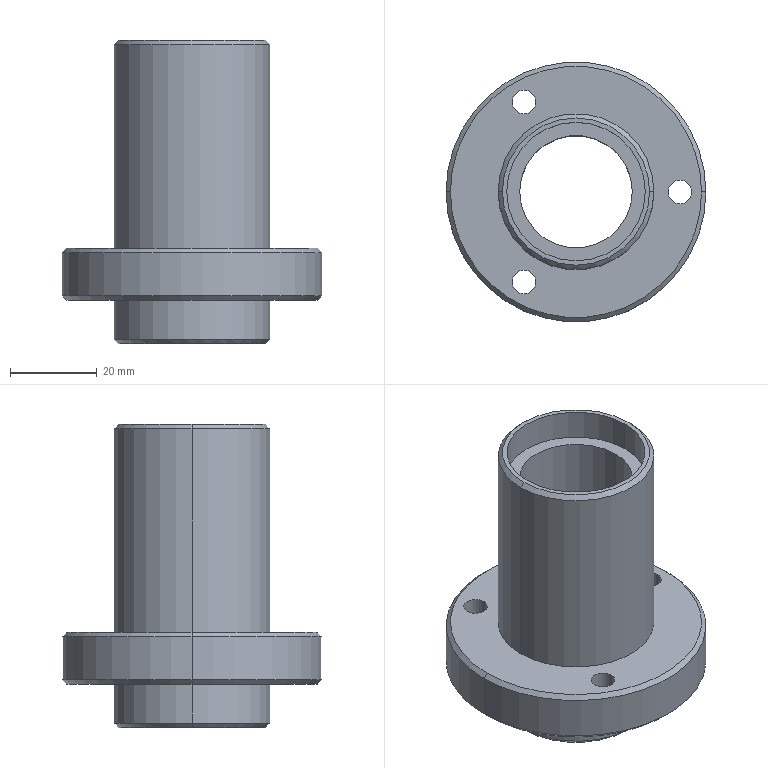Component | SolidWorks | JYTBJ-HeaderPlateFlangeSeatA-1 | 1 solid | 32 faces | box 60 x 60 x 70 mm | volume 50822 mm3 | cylinder 18 | cone 8 | plane 6 | commonest cylinder face diameters 5.5 x6 32 x4 36 x4 26 x2 60 x2
build123d program:
from build123d import *

# Parameters (mm, degrees)
F_5_5_5_5_DIAMETER_HOLE1_D = 5.5
CIRPATTERN1_COUNT          = 3
CHAMFER1_SIZE              = 1


with BuildPart() as part:
    # Sketch1 → Revolve1 (revolve)
    with BuildSketch(Plane.XY, mode=Mode.PRIVATE) as revolve1_sk:
        Polygon((16, 0), (18, 0), (18, 48), (30, 48), (30, 60), (18, 60), (18, 70), (16, 70), (16, 63), (13, 63), (13, 7), (16, 7), align=None)
    revolve(revolve1_sk.sketch.rotate(Axis((0, 0, 0), (0, 1, 0)), 90), axis=Axis((0, 0, 0), (0, 1, 0)))

    # 5.5 _5.5_ Diameter Hole1 (through all)
    with Locations(Plane.XZ.offset(-48)):
        with Locations((0, 24)):
            f_5_5_5_5_diameter_hole1 = Hole(F_5_5_5_5_DIAMETER_HOLE1_D / 2)

    # CirPattern1: 5.5 _5.5_ Diameter Hole1 ×3 about axis
    cirpattern1_axis = Axis((0, 0, 0), (0, 1, 0))
    for i in range(1, CIRPATTERN1_COUNT):
        add(f_5_5_5_5_diameter_hole1.rotate(cirpattern1_axis, i * 360 / CIRPATTERN1_COUNT), mode=Mode.SUBTRACT)

    # Chamfer1
    chamfer1_edges = [part.edges().sort_by_distance(p)[0] for p in [
        (0, 70, 18),
        (0, 60, 30),
        (0, 48, 30),
        (0, 0, 18),
    ]]
    chamfer(chamfer1_edges, length=CHAMFER1_SIZE)


solid = part.part

# Placed as in the assembly
solid = solid.moved(Location((3.373, 96.878, 42), (-90, 90, 0)))
STEP:
#1=COLOUR_RGB('',0.7922,0.8196,0.9333);
#2=FILL_AREA_STYLE_COLOUR('',#1);
#3=FILL_AREA_STYLE('',(#2));
#4=SURFACE_STYLE_FILL_AREA(#3);
#5=SURFACE_SIDE_STYLE('',(#4));
#6=SURFACE_STYLE_USAGE(.BOTH.,#5);
#7=PRESENTATION_STYLE_ASSIGNMENT((#6));
#8=CARTESIAN_POINT('',(-0.5365,3.814,1.654));
#9=VERTEX_POINT('',#8);
#10=CARTESIAN_POINT('',(0.8021,3.814,1.654));
#11=VERTEX_POINT('',#10);
#12=CARTESIAN_POINT('',(0.1328,3.814,1.654));
#13=DIRECTION('',(0.,0.,1.));
#14=DIRECTION('',(-1.,0.,0.));
#15=AXIS2_PLACEMENT_3D('',#12,#13,#14);
#16=CIRCLE('',#15,0.6693);
#17=EDGE_CURVE('',#9,#11,#16,.T.);
#18=ORIENTED_EDGE('',*,*,#17,.F.);
#19=CARTESIAN_POINT('',(-0.5759,3.814,1.614));
#20=VERTEX_POINT('',#19);
#21=CARTESIAN_POINT('',(-0.5365,3.814,1.654));
#22=DIRECTION('',(-0.7071,-0.,-0.7071));
#23=VECTOR('',#22,39.37);
#24=LINE('',#21,#23);
#25=EDGE_CURVE('',#9,#20,#24,.T.);
#26=ORIENTED_EDGE('',*,*,#25,.T.);
#27=CARTESIAN_POINT('',(0.8415,3.814,1.614));
#28=VERTEX_POINT('',#27);
#29=CARTESIAN_POINT('',(0.1328,3.814,1.614));
#30=DIRECTION('',(0.,0.,-1.));
#31=DIRECTION('',(-1.,0.,0.));
#32=AXIS2_PLACEMENT_3D('',#29,#30,#31);
#33=CIRCLE('',#32,0.7087);
#34=EDGE_CURVE('',#28,#20,#33,.T.);
#35=ORIENTED_EDGE('',*,*,#34,.F.);
#36=CARTESIAN_POINT('',(0.8021,3.814,1.654));
#37=DIRECTION('',(0.7071,-0.,-0.7071));
#38=VECTOR('',#37,39.37);
#39=LINE('',#36,#38);
#40=EDGE_CURVE('',#11,#28,#39,.T.);
#41=ORIENTED_EDGE('',*,*,#40,.F.);
#42=EDGE_LOOP('',(#18,#26,#35,#41));
#43=FACE_OUTER_BOUND('',#42,.T.);
#44=CARTESIAN_POINT('',(0.1328,3.814,1.654));
#45=DIRECTION('',(0.,0.,-1.));
#46=DIRECTION('',(1.,0.,0.));
#47=AXIS2_PLACEMENT_3D('',#44,#45,#46);
#48=CONICAL_SURFACE('',#47,0.6693,0.7854);
#49=ADVANCED_FACE('',(#43),#48,.T.);
#50=CARTESIAN_POINT('',(-1.009,3.814,-0.2362));
#51=VERTEX_POINT('',#50);
#52=CARTESIAN_POINT('',(1.275,3.814,-0.2362));
#53=VERTEX_POINT('',#52);
#54=CARTESIAN_POINT('',(0.1328,3.814,-0.2362));
#55=DIRECTION('',(0.,0.,1.));
#56=DIRECTION('',(-1.,0.,0.));
#57=AXIS2_PLACEMENT_3D('',#54,#55,#56);
#58=CIRCLE('',#57,1.142);
#59=EDGE_CURVE('',#51,#53,#58,.T.);
#60=ORIENTED_EDGE('',*,*,#59,.F.);
#61=CARTESIAN_POINT('',(-1.048,3.814,-0.2756));
#62=VERTEX_POINT('',#61);
#63=CARTESIAN_POINT('',(-1.009,3.814,-0.2362));
#64=DIRECTION('',(-0.7071,-0.,-0.7071));
#65=VECTOR('',#64,39.37);
#66=LINE('',#63,#65);
#67=EDGE_CURVE('',#51,#62,#66,.T.);
#68=ORIENTED_EDGE('',*,*,#67,.T.);
#69=CARTESIAN_POINT('',(1.314,3.814,-0.2756));
#70=VERTEX_POINT('',#69);
#71=CARTESIAN_POINT('',(0.1328,3.814,-0.2756));
#72=DIRECTION('',(0.,0.,-1.));
#73=DIRECTION('',(-1.,0.,0.));
#74=AXIS2_PLACEMENT_3D('',#71,#72,#73);
#75=CIRCLE('',#74,1.181);
#76=EDGE_CURVE('',#70,#62,#75,.T.);
#77=ORIENTED_EDGE('',*,*,#76,.F.);
#78=CARTESIAN_POINT('',(1.275,3.814,-0.2362));
#79=DIRECTION('',(0.7071,-0.,-0.7071));
#80=VECTOR('',#79,39.37);
#81=LINE('',#78,#80);
#82=EDGE_CURVE('',#53,#70,#81,.T.);
#83=ORIENTED_EDGE('',*,*,#82,.F.);
#84=EDGE_LOOP('',(#60,#68,#77,#83));
#85=FACE_OUTER_BOUND('',#84,.T.);
#86=CARTESIAN_POINT('',(0.1328,3.814,-0.2362));
#87=DIRECTION('',(0.,0.,-1.));
#88=DIRECTION('',(1.,0.,0.));
#89=AXIS2_PLACEMENT_3D('',#86,#87,#88);
#90=CONICAL_SURFACE('',#89,1.142,0.7854);
#91=ADVANCED_FACE('',(#85),#90,.T.);
#92=CARTESIAN_POINT('',(1.275,3.814,-0.7087));
#93=VERTEX_POINT('',#92);
#94=CARTESIAN_POINT('',(-1.009,3.814,-0.7087));
#95=VERTEX_POINT('',#94);
#96=CARTESIAN_POINT('',(0.1328,3.814,-0.7087));
#97=DIRECTION('',(0.,0.,-1.));
#98=DIRECTION('',(1.,0.,0.));
#99=AXIS2_PLACEMENT_3D('',#96,#97,#98);
#100=CIRCLE('',#99,1.142);
#101=EDGE_CURVE('',#93,#95,#100,.T.);
#102=ORIENTED_EDGE('',*,*,#101,.F.);
#103=CARTESIAN_POINT('',(1.314,3.814,-0.6693));
#104=VERTEX_POINT('',#103);
#105=CARTESIAN_POINT('',(1.314,3.814,-0.6693));
#106=DIRECTION('',(0.7071,-0.,0.7071));
#107=VECTOR('',#106,39.37);
#108=LINE('',#105,#107);
#109=EDGE_CURVE('',#93,#104,#108,.T.);
#110=ORIENTED_EDGE('',*,*,#109,.T.);
#111=CARTESIAN_POINT('',(-1.048,3.814,-0.6693));
#112=VERTEX_POINT('',#111);
#113=CARTESIAN_POINT('',(0.1328,3.814,-0.6693));
#114=DIRECTION('',(0.,0.,1.));
#115=DIRECTION('',(1.,0.,0.));
#116=AXIS2_PLACEMENT_3D('',#113,#114,#115);
#117=CIRCLE('',#116,1.181);
#118=EDGE_CURVE('',#112,#104,#117,.T.);
#119=ORIENTED_EDGE('',*,*,#118,.F.);
#120=CARTESIAN_POINT('',(-1.048,3.814,-0.6693));
#121=DIRECTION('',(-0.7071,0.,0.7071));
#122=VECTOR('',#121,39.37);
#123=LINE('',#120,#122);
#124=EDGE_CURVE('',#95,#112,#123,.T.);
#125=ORIENTED_EDGE('',*,*,#124,.F.);
#126=EDGE_LOOP('',(#102,#110,#119,#125));
#127=FACE_OUTER_BOUND('',#126,.T.);
#128=CARTESIAN_POINT('',(0.1328,3.814,-0.6693));
#129=DIRECTION('',(0.,0.,1.));
#130=DIRECTION('',(-1.,0.,0.));
#131=AXIS2_PLACEMENT_3D('',#128,#129,#130);
#132=CONICAL_SURFACE('',#131,1.181,0.7854);
#133=ADVANCED_FACE('',(#127),#132,.T.);
#134=CARTESIAN_POINT('',(0.8021,3.814,-1.102));
#135=VERTEX_POINT('',#134);
#136=CARTESIAN_POINT('',(-0.5365,3.814,-1.102));
#137=VERTEX_POINT('',#136);
#138=CARTESIAN_POINT('',(0.1328,3.814,-1.102));
#139=DIRECTION('',(0.,0.,-1.));
#140=DIRECTION('',(1.,0.,0.));
#141=AXIS2_PLACEMENT_3D('',#138,#139,#140);
#142=CIRCLE('',#141,0.6693);
#143=EDGE_CURVE('',#135,#137,#142,.T.);
#144=ORIENTED_EDGE('',*,*,#143,.F.);
#145=CARTESIAN_POINT('',(0.8415,3.814,-1.063));
#146=VERTEX_POINT('',#145);
#147=CARTESIAN_POINT('',(0.8415,3.814,-1.063));
#148=DIRECTION('',(0.7071,-0.,0.7071));
#149=VECTOR('',#148,39.37);
#150=LINE('',#147,#149);
#151=EDGE_CURVE('',#135,#146,#150,.T.);
#152=ORIENTED_EDGE('',*,*,#151,.T.);
#153=CARTESIAN_POINT('',(-0.5759,3.814,-1.063));
#154=VERTEX_POINT('',#153);
#155=CARTESIAN_POINT('',(0.1328,3.814,-1.063));
#156=DIRECTION('',(0.,0.,1.));
#157=DIRECTION('',(1.,0.,0.));
#158=AXIS2_PLACEMENT_3D('',#155,#156,#157);
#159=CIRCLE('',#158,0.7087);
#160=EDGE_CURVE('',#154,#146,#159,.T.);
#161=ORIENTED_EDGE('',*,*,#160,.F.);
#162=CARTESIAN_POINT('',(-0.5759,3.814,-1.063));
#163=DIRECTION('',(-0.7071,0.,0.7071));
#164=VECTOR('',#163,39.37);
#165=LINE('',#162,#164);
#166=EDGE_CURVE('',#137,#154,#165,.T.);
#167=ORIENTED_EDGE('',*,*,#166,.F.);
#168=EDGE_LOOP('',(#144,#152,#161,#167));
#169=FACE_OUTER_BOUND('',#168,.T.);
#170=CARTESIAN_POINT('',(0.1328,3.814,-1.063));
#171=DIRECTION('',(0.,0.,1.));
#172=DIRECTION('',(-1.,0.,0.));
#173=AXIS2_PLACEMENT_3D('',#170,#171,#172);
#174=CONICAL_SURFACE('',#173,0.7087,0.7854);
#175=ADVANCED_FACE('',(#169),#174,.T.);
#176=CARTESIAN_POINT('',(-0.4479,2.996,-0.7087));
#177=VERTEX_POINT('',#176);
#178=CARTESIAN_POINT('',(-0.2314,2.996,-0.7087));
#179=VERTEX_POINT('',#178);
#180=CARTESIAN_POINT('',(-0.3396,2.996,-0.7087));
#181=DIRECTION('',(0.,0.,-1.));
#182=DIRECTION('',(1.,0.,0.));
#183=AXIS2_PLACEMENT_3D('',#180,#181,#182);
#184=CIRCLE('',#183,0.1083);
#185=EDGE_CURVE('',#177,#179,#184,.T.);
#186=ORIENTED_EDGE('',*,*,#185,.T.);
#187=CARTESIAN_POINT('',(-0.2314,2.996,-0.2362));
#188=VERTEX_POINT('',#187);
#189=CARTESIAN_POINT('',(-0.2314,2.996,-0.2362));
#190=DIRECTION('',(0.,0.,1.));
#191=VECTOR('',#190,39.37);
#192=LINE('',#189,#191);
#193=EDGE_CURVE('',#179,#188,#192,.T.);
#194=ORIENTED_EDGE('',*,*,#193,.T.);
#195=CARTESIAN_POINT('',(-0.4479,2.996,-0.2362));
#196=VERTEX_POINT('',#195);
#197=CARTESIAN_POINT('',(-0.3396,2.996,-0.2362));
#198=DIRECTION('',(0.,0.,1.));
#199=DIRECTION('',(-1.,0.,0.));
#200=AXIS2_PLACEMENT_3D('',#197,#198,#199);
#201=CIRCLE('',#200,0.1083);
#202=EDGE_CURVE('',#188,#196,#201,.T.);
#203=ORIENTED_EDGE('',*,*,#202,.T.);
#204=CARTESIAN_POINT('',(-0.4479,2.996,-0.2362));
#205=DIRECTION('',(0.,0.,1.));
#206=VECTOR('',#205,39.37);
#207=LINE('',#204,#206);
#208=EDGE_CURVE('',#177,#196,#207,.T.);
#209=ORIENTED_EDGE('',*,*,#208,.F.);
#210=EDGE_LOOP('',(#186,#194,#203,#209));
#211=FACE_OUTER_BOUND('',#210,.T.);
#212=CARTESIAN_POINT('',(-0.3396,2.996,-0.2362));
#213=DIRECTION('',(0.,0.,1.));
#214=DIRECTION('',(-1.,0.,0.));
#215=AXIS2_PLACEMENT_3D('',#212,#213,#214);
#216=CYLINDRICAL_SURFACE('',#215,0.1083);
#217=ADVANCED_FACE('',(#211),#216,.F.);
#218=CARTESIAN_POINT('',(-0.4479,4.632,-0.7087));
#219=VERTEX_POINT('',#218);
#220=CARTESIAN_POINT('',(-0.2314,4.632,-0.7087));
#221=VERTEX_POINT('',#220);
#222=CARTESIAN_POINT('',(-0.3396,4.632,-0.7087));
#223=DIRECTION('',(0.,0.,-1.));
#224=DIRECTION('',(1.,0.,0.));
#225=AXIS2_PLACEMENT_3D('',#222,#223,#224);
#226=CIRCLE('',#225,0.1083);
#227=EDGE_CURVE('',#219,#221,#226,.T.);
#228=ORIENTED_EDGE('',*,*,#227,.T.);
#229=CARTESIAN_POINT('',(-0.2314,4.632,-0.2362));
#230=VERTEX_POINT('',#229);
#231=CARTESIAN_POINT('',(-0.2314,4.632,-0.2362));
#232=DIRECTION('',(0.,0.,1.));
#233=VECTOR('',#232,39.37);
#234=LINE('',#231,#233);
#235=EDGE_CURVE('',#221,#230,#234,.T.);
#236=ORIENTED_EDGE('',*,*,#235,.T.);
#237=CARTESIAN_POINT('',(-0.4479,4.632,-0.2362));
#238=VERTEX_POINT('',#237);
#239=CARTESIAN_POINT('',(-0.3396,4.632,-0.2362));
#240=DIRECTION('',(0.,0.,1.));
#241=DIRECTION('',(-1.,0.,0.));
#242=AXIS2_PLACEMENT_3D('',#239,#240,#241);
#243=CIRCLE('',#242,0.1083);
#244=EDGE_CURVE('',#230,#238,#243,.T.);
#245=ORIENTED_EDGE('',*,*,#244,.T.);
#246=CARTESIAN_POINT('',(-0.4479,4.632,-0.2362));
#247=DIRECTION('',(0.,0.,1.));
#248=VECTOR('',#247,39.37);
#249=LINE('',#246,#248);
#250=EDGE_CURVE('',#219,#238,#249,.T.);
#251=ORIENTED_EDGE('',*,*,#250,.F.);
#252=EDGE_LOOP('',(#228,#236,#245,#251));
#253=FACE_OUTER_BOUND('',#252,.T.);
#254=CARTESIAN_POINT('',(-0.3396,4.632,-0.2362));
#255=DIRECTION('',(0.,0.,1.));
#256=DIRECTION('',(-1.,0.,0.));
#257=AXIS2_PLACEMENT_3D('',#254,#255,#256);
#258=CYLINDRICAL_SURFACE('',#257,0.1083);
#259=ADVANCED_FACE('',(#253),#258,.F.);
#260=CARTESIAN_POINT('',(0.9694,3.814,-0.7087));
#261=VERTEX_POINT('',#260);
#262=CARTESIAN_POINT('',(1.186,3.814,-0.7087));
#263=VERTEX_POINT('',#262);
#264=CARTESIAN_POINT('',(1.078,3.814,-0.7087));
#265=DIRECTION('',(0.,0.,-1.));
#266=DIRECTION('',(1.,0.,0.));
#267=AXIS2_PLACEMENT_3D('',#264,#265,#266);
#268=CIRCLE('',#267,0.1083);
#269=EDGE_CURVE('',#261,#263,#268,.T.);
#270=ORIENTED_EDGE('',*,*,#269,.T.);
#271=CARTESIAN_POINT('',(1.186,3.814,-0.2362));
#272=VERTEX_POINT('',#271);
#273=CARTESIAN_POINT('',(1.186,3.814,-0.2362));
#274=DIRECTION('',(0.,0.,1.));
#275=VECTOR('',#274,39.37);
#276=LINE('',#273,#275);
#277=EDGE_CURVE('',#263,#272,#276,.T.);
#278=ORIENTED_EDGE('',*,*,#277,.T.);
#279=CARTESIAN_POINT('',(0.9694,3.814,-0.2362));
#280=VERTEX_POINT('',#279);
#281=CARTESIAN_POINT('',(1.078,3.814,-0.2362));
#282=DIRECTION('',(0.,0.,1.));
#283=DIRECTION('',(-1.,0.,0.));
#284=AXIS2_PLACEMENT_3D('',#281,#282,#283);
#285=CIRCLE('',#284,0.1083);
#286=EDGE_CURVE('',#272,#280,#285,.T.);
#287=ORIENTED_EDGE('',*,*,#286,.T.);
#288=CARTESIAN_POINT('',(0.9694,3.814,-0.2362));
#289=DIRECTION('',(0.,0.,1.));
#290=VECTOR('',#289,39.37);
#291=LINE('',#288,#290);
#292=EDGE_CURVE('',#261,#280,#291,.T.);
#293=ORIENTED_EDGE('',*,*,#292,.F.);
#294=EDGE_LOOP('',(#270,#278,#287,#293));
#295=FACE_OUTER_BOUND('',#294,.T.);
#296=CARTESIAN_POINT('',(1.078,3.814,-0.2362));
#297=DIRECTION('',(0.,0.,1.));
#298=DIRECTION('',(-1.,0.,0.));
#299=AXIS2_PLACEMENT_3D('',#296,#297,#298);
#300=CYLINDRICAL_SURFACE('',#299,0.1083);
#301=ADVANCED_FACE('',(#295),#300,.F.);
#302=CARTESIAN_POINT('',(0.6446,3.814,-0.8268));
#303=VERTEX_POINT('',#302);
#304=CARTESIAN_POINT('',(-0.379,3.814,-0.8268));
#305=VERTEX_POINT('',#304);
#306=CARTESIAN_POINT('',(0.1328,3.814,-0.8268));
#307=DIRECTION('',(0.,0.,1.));
#308=DIRECTION('',(-1.,0.,0.));
#309=AXIS2_PLACEMENT_3D('',#306,#307,#308);
#310=CIRCLE('',#309,0.5118);
#311=EDGE_CURVE('',#303,#305,#310,.T.);
#312=ORIENTED_EDGE('',*,*,#311,.F.);
#313=CARTESIAN_POINT('',(0.6446,3.814,1.378));
#314=VERTEX_POINT('',#313);
#315=CARTESIAN_POINT('',(0.6446,3.814,1.654));
#316=DIRECTION('',(0.,0.,1.));
#317=VECTOR('',#316,39.37);
#318=LINE('',#315,#317);
#319=EDGE_CURVE('',#303,#314,#318,.T.);
#320=ORIENTED_EDGE('',*,*,#319,.T.);
#321=CARTESIAN_POINT('',(-0.379,3.814,1.378));
#322=VERTEX_POINT('',#321);
#323=CARTESIAN_POINT('',(0.1328,3.814,1.378));
#324=DIRECTION('',(0.,0.,1.));
#325=DIRECTION('',(-1.,0.,0.));
#326=AXIS2_PLACEMENT_3D('',#323,#324,#325);
#327=CIRCLE('',#326,0.5118);
#328=EDGE_CURVE('',#314,#322,#327,.T.);
#329=ORIENTED_EDGE('',*,*,#328,.T.);
#330=CARTESIAN_POINT('',(-0.379,3.814,1.654));
#331=DIRECTION('',(0.,0.,1.));
#332=VECTOR('',#331,39.37);
#333=LINE('',#330,#332);
#334=EDGE_CURVE('',#305,#322,#333,.T.);
#335=ORIENTED_EDGE('',*,*,#334,.F.);
#336=EDGE_LOOP('',(#312,#320,#329,#335));
#337=FACE_OUTER_BOUND('',#336,.T.);
#338=CARTESIAN_POINT('',(0.1328,3.814,1.654));
#339=DIRECTION('',(0.,0.,1.));
#340=DIRECTION('',(-1.,0.,0.));
#341=AXIS2_PLACEMENT_3D('',#338,#339,#340);
#342=CYLINDRICAL_SURFACE('',#341,0.5118);
#343=ADVANCED_FACE('',(#337),#342,.F.);
#344=CARTESIAN_POINT('',(0.7627,3.814,-1.102));
#345=VERTEX_POINT('',#344);
#346=CARTESIAN_POINT('',(-0.4971,3.814,-1.102));
#347=VERTEX_POINT('',#346);
#348=CARTESIAN_POINT('',(0.1328,3.814,-1.102));
#349=DIRECTION('',(0.,0.,1.));
#350=DIRECTION('',(-1.,0.,0.));
#351=AXIS2_PLACEMENT_3D('',#348,#349,#350);
#352=CIRCLE('',#351,0.6299);
#353=EDGE_CURVE('',#345,#347,#352,.T.);
#354=ORIENTED_EDGE('',*,*,#353,.F.);
#355=CARTESIAN_POINT('',(0.7627,3.814,-0.8268));
#356=VERTEX_POINT('',#355);
#357=CARTESIAN_POINT('',(0.7627,3.814,1.654));
#358=DIRECTION('',(0.,0.,1.));
#359=VECTOR('',#358,39.37);
#360=LINE('',#357,#359);
#361=EDGE_CURVE('',#345,#356,#360,.T.);
#362=ORIENTED_EDGE('',*,*,#361,.T.);
#363=CARTESIAN_POINT('',(-0.4971,3.814,-0.8268));
#364=VERTEX_POINT('',#363);
#365=CARTESIAN_POINT('',(0.1328,3.814,-0.8268));
#366=DIRECTION('',(0.,0.,1.));
#367=DIRECTION('',(-1.,0.,0.));
#368=AXIS2_PLACEMENT_3D('',#365,#366,#367);
#369=CIRCLE('',#368,0.6299);
#370=EDGE_CURVE('',#356,#364,#369,.T.);
#371=ORIENTED_EDGE('',*,*,#370,.T.);
#372=CARTESIAN_POINT('',(-0.4971,3.814,1.654));
#373=DIRECTION('',(0.,0.,1.));
#374=VECTOR('',#373,39.37);
#375=LINE('',#372,#374);
#376=EDGE_CURVE('',#347,#364,#375,.T.);
#377=ORIENTED_EDGE('',*,*,#376,.F.);
#378=EDGE_LOOP('',(#354,#362,#371,#377));
#379=FACE_OUTER_BOUND('',#378,.T.);
#380=CARTESIAN_POINT('',(0.1328,3.814,1.654));
#381=DIRECTION('',(0.,0.,1.));
#382=DIRECTION('',(-1.,0.,0.));
#383=AXIS2_PLACEMENT_3D('',#380,#381,#382);
#384=CYLINDRICAL_SURFACE('',#383,0.6299);
#385=ADVANCED_FACE('',(#379),#384,.F.);
#386=ORIENTED_EDGE('',*,*,#160,.T.);
#387=CARTESIAN_POINT('',(0.8415,3.814,-0.7087));
#388=VERTEX_POINT('',#387);
#389=CARTESIAN_POINT('',(0.8415,3.814,1.654));
#390=DIRECTION('',(0.,0.,1.));
#391=VECTOR('',#390,39.37);
#392=LINE('',#389,#391);
#393=EDGE_CURVE('',#146,#388,#392,.T.);
#394=ORIENTED_EDGE('',*,*,#393,.T.);
#395=CARTESIAN_POINT('',(-0.5759,3.814,-0.7087));
#396=VERTEX_POINT('',#395);
#397=CARTESIAN_POINT('',(0.1328,3.814,-0.7087));
#398=DIRECTION('',(0.,0.,1.));
#399=DIRECTION('',(-1.,0.,0.));
#400=AXIS2_PLACEMENT_3D('',#397,#398,#399);
#401=CIRCLE('',#400,0.7087);
#402=EDGE_CURVE('',#396,#388,#401,.T.);
#403=ORIENTED_EDGE('',*,*,#402,.F.);
#404=CARTESIAN_POINT('',(-0.5759,3.814,1.654));
#405=DIRECTION('',(0.,0.,1.));
#406=VECTOR('',#405,39.37);
#407=LINE('',#404,#406);
#408=EDGE_CURVE('',#154,#396,#407,.T.);
#409=ORIENTED_EDGE('',*,*,#408,.F.);
#410=EDGE_LOOP('',(#386,#394,#403,#409));
#411=FACE_OUTER_BOUND('',#410,.T.);
#412=CARTESIAN_POINT('',(0.1328,3.814,1.654));
#413=DIRECTION('',(0.,0.,1.));
#414=DIRECTION('',(-1.,0.,0.));
#415=AXIS2_PLACEMENT_3D('',#412,#413,#414);
#416=CYLINDRICAL_SURFACE('',#415,0.7087);
#417=ADVANCED_FACE('',(#411),#416,.T.);
#418=ORIENTED_EDGE('',*,*,#118,.T.);
#419=CARTESIAN_POINT('',(1.314,3.814,1.654));
#420=DIRECTION('',(0.,0.,1.));
#421=VECTOR('',#420,39.37);
#422=LINE('',#419,#421);
#423=EDGE_CURVE('',#104,#70,#422,.T.);
#424=ORIENTED_EDGE('',*,*,#423,.T.);
#425=ORIENTED_EDGE('',*,*,#76,.T.);
#426=CARTESIAN_POINT('',(-1.048,3.814,1.654));
#427=DIRECTION('',(0.,0.,1.));
#428=VECTOR('',#427,39.37);
#429=LINE('',#426,#428);
#430=EDGE_CURVE('',#112,#62,#429,.T.);
#431=ORIENTED_EDGE('',*,*,#430,.F.);
#432=EDGE_LOOP('',(#418,#424,#425,#431));
#433=FACE_OUTER_BOUND('',#432,.T.);
#434=CARTESIAN_POINT('',(0.1328,3.814,1.654));
#435=DIRECTION('',(0.,0.,1.));
#436=DIRECTION('',(-1.,0.,0.));
#437=AXIS2_PLACEMENT_3D('',#434,#435,#436);
#438=CYLINDRICAL_SURFACE('',#437,1.181);
#439=ADVANCED_FACE('',(#433),#438,.T.);
#440=CARTESIAN_POINT('',(-0.5759,3.814,-0.2362));
#441=VERTEX_POINT('',#440);
#442=CARTESIAN_POINT('',(0.8415,3.814,-0.2362));
#443=VERTEX_POINT('',#442);
#444=CARTESIAN_POINT('',(0.1328,3.814,-0.2362));
#445=DIRECTION('',(0.,0.,1.));
#446=DIRECTION('',(-1.,0.,0.));
#447=AXIS2_PLACEMENT_3D('',#444,#445,#446);
#448=CIRCLE('',#447,0.7087);
#449=EDGE_CURVE('',#441,#443,#448,.T.);
#450=ORIENTED_EDGE('',*,*,#449,.T.);
#451=CARTESIAN_POINT('',(0.8415,3.814,1.654));
#452=DIRECTION('',(0.,0.,1.));
#453=VECTOR('',#452,39.37);
#454=LINE('',#451,#453);
#455=EDGE_CURVE('',#443,#28,#454,.T.);
#456=ORIENTED_EDGE('',*,*,#455,.T.);
#457=ORIENTED_EDGE('',*,*,#34,.T.);
#458=CARTESIAN_POINT('',(-0.5759,3.814,1.654));
#459=DIRECTION('',(0.,0.,1.));
#460=VECTOR('',#459,39.37);
#461=LINE('',#458,#460);
#462=EDGE_CURVE('',#441,#20,#461,.T.);
#463=ORIENTED_EDGE('',*,*,#462,.F.);
#464=EDGE_LOOP('',(#450,#456,#457,#463));
#465=FACE_OUTER_BOUND('',#464,.T.);
#466=CARTESIAN_POINT('',(0.1328,3.814,1.654));
#467=DIRECTION('',(0.,0.,1.));
#468=DIRECTION('',(-1.,0.,0.));
#469=AXIS2_PLACEMENT_3D('',#466,#467,#468);
#470=CYLINDRICAL_SURFACE('',#469,0.7087);
#471=ADVANCED_FACE('',(#465),#470,.T.);
#472=CARTESIAN_POINT('',(0.7627,3.814,1.378));
#473=VERTEX_POINT('',#472);
#474=CARTESIAN_POINT('',(-0.4971,3.814,1.378));
#475=VERTEX_POINT('',#474);
#476=CARTESIAN_POINT('',(0.1328,3.814,1.378));
#477=DIRECTION('',(0.,0.,1.));
#478=DIRECTION('',(-1.,0.,0.));
#479=AXIS2_PLACEMENT_3D('',#476,#477,#478);
#480=CIRCLE('',#479,0.6299);
#481=EDGE_CURVE('',#473,#475,#480,.T.);
#482=ORIENTED_EDGE('',*,*,#481,.F.);
#483=CARTESIAN_POINT('',(0.7627,3.814,1.654));
#484=VERTEX_POINT('',#483);
#485=CARTESIAN_POINT('',(0.7627,3.814,1.654));
#486=DIRECTION('',(0.,0.,1.));
#487=VECTOR('',#486,39.37);
#488=LINE('',#485,#487);
#489=EDGE_CURVE('',#473,#484,#488,.T.);
#490=ORIENTED_EDGE('',*,*,#489,.T.);
#491=CARTESIAN_POINT('',(-0.4971,3.814,1.654));
#492=VERTEX_POINT('',#491);
#493=CARTESIAN_POINT('',(0.1328,3.814,1.654));
#494=DIRECTION('',(0.,0.,1.));
#495=DIRECTION('',(-1.,0.,0.));
#496=AXIS2_PLACEMENT_3D('',#493,#494,#495);
#497=CIRCLE('',#496,0.6299);
#498=EDGE_CURVE('',#484,#492,#497,.T.);
#499=ORIENTED_EDGE('',*,*,#498,.T.);
#500=CARTESIAN_POINT('',(-0.4971,3.814,1.654));
#501=DIRECTION('',(0.,0.,1.));
#502=VECTOR('',#501,39.37);
#503=LINE('',#500,#502);
#504=EDGE_CURVE('',#475,#492,#503,.T.);
#505=ORIENTED_EDGE('',*,*,#504,.F.);
#506=EDGE_LOOP('',(#482,#490,#499,#505));
#507=FACE_OUTER_BOUND('',#506,.T.);
#508=CARTESIAN_POINT('',(0.1328,3.814,1.654));
#509=DIRECTION('',(0.,0.,1.));
#510=DIRECTION('',(-1.,0.,0.));
#511=AXIS2_PLACEMENT_3D('',#508,#509,#510);
#512=CYLINDRICAL_SURFACE('',#511,0.6299);
#513=ADVANCED_FACE('',(#507),#512,.F.);
#514=ORIENTED_EDGE('',*,*,#489,.F.);
#515=CARTESIAN_POINT('',(0.1328,3.814,1.378));
#516=DIRECTION('',(0.,0.,1.));
#517=DIRECTION('',(-1.,0.,0.));
#518=AXIS2_PLACEMENT_3D('',#515,#516,#517);
#519=CIRCLE('',#518,0.6299);
#520=EDGE_CURVE('',#475,#473,#519,.T.);
#521=ORIENTED_EDGE('',*,*,#520,.F.);
#522=ORIENTED_EDGE('',*,*,#504,.T.);
#523=CARTESIAN_POINT('',(0.1328,3.814,1.654));
#524=DIRECTION('',(0.,0.,1.));
#525=DIRECTION('',(-1.,0.,0.));
#526=AXIS2_PLACEMENT_3D('',#523,#524,#525);
#527=CIRCLE('',#526,0.6299);
#528=EDGE_CURVE('',#492,#484,#527,.T.);
#529=ORIENTED_EDGE('',*,*,#528,.T.);
#530=EDGE_LOOP('',(#514,#521,#522,#529));
#531=FACE_OUTER_BOUND('',#530,.T.);
#532=CARTESIAN_POINT('',(0.1328,3.814,1.654));
#533=DIRECTION('',(0.,0.,1.));
#534=DIRECTION('',(-1.,0.,0.));
#535=AXIS2_PLACEMENT_3D('',#532,#533,#534);
#536=CYLINDRICAL_SURFACE('',#535,0.6299);
#537=ADVANCED_FACE('',(#531),#536,.F.);
#538=CARTESIAN_POINT('',(0.1328,3.814,1.654));
#539=DIRECTION('',(0.,0.,1.));
#540=DIRECTION('',(-1.,0.,0.));
#541=AXIS2_PLACEMENT_3D('',#538,#539,#540);
#542=CIRCLE('',#541,0.6693);
#543=EDGE_CURVE('',#11,#9,#542,.T.);
#544=ORIENTED_EDGE('',*,*,#543,.T.);
#545=ORIENTED_EDGE('',*,*,#17,.T.);
#546=EDGE_LOOP('',(#544,#545));
#547=FACE_OUTER_BOUND('',#546,.T.);
#548=ORIENTED_EDGE('',*,*,#528,.F.);
#549=ORIENTED_EDGE('',*,*,#498,.F.);
#550=EDGE_LOOP('',(#548,#549));
#551=FACE_BOUND('',#550,.T.);
#552=CARTESIAN_POINT('',(0.1328,3.184,1.654));
#553=DIRECTION('',(0.,0.,1.));
#554=DIRECTION('',(-1.,0.,0.));
#555=AXIS2_PLACEMENT_3D('',#552,#553,#554);
#556=PLANE('',#555);
#557=ADVANCED_FACE('',(#547,#551),#556,.T.);
#558=ORIENTED_EDGE('',*,*,#455,.F.);
#559=CARTESIAN_POINT('',(0.1328,3.814,-0.2362));
#560=DIRECTION('',(0.,0.,1.));
#561=DIRECTION('',(-1.,0.,0.));
#562=AXIS2_PLACEMENT_3D('',#559,#560,#561);
#563=CIRCLE('',#562,0.7087);
#564=EDGE_CURVE('',#443,#441,#563,.T.);
#565=ORIENTED_EDGE('',*,*,#564,.T.);
#566=ORIENTED_EDGE('',*,*,#462,.T.);
#567=CARTESIAN_POINT('',(0.1328,3.814,1.614));
#568=DIRECTION('',(0.,0.,-1.));
#569=DIRECTION('',(-1.,0.,0.));
#570=AXIS2_PLACEMENT_3D('',#567,#568,#569);
#571=CIRCLE('',#570,0.7087);
#572=EDGE_CURVE('',#20,#28,#571,.T.);
#573=ORIENTED_EDGE('',*,*,#572,.T.);
#574=EDGE_LOOP('',(#558,#565,#566,#573));
#575=FACE_OUTER_BOUND('',#574,.T.);
#576=CARTESIAN_POINT('',(0.1328,3.814,1.654));
#577=DIRECTION('',(0.,0.,1.));
#578=DIRECTION('',(-1.,0.,0.));
#579=AXIS2_PLACEMENT_3D('',#576,#577,#578);
#580=CYLINDRICAL_SURFACE('',#579,0.7087);
#581=ADVANCED_FACE('',(#575),#580,.T.);
#582=CARTESIAN_POINT('',(0.1328,3.814,-0.2362));
#583=DIRECTION('',(0.,0.,1.));
#584=DIRECTION('',(-1.,0.,0.));
#585=AXIS2_PLACEMENT_3D('',#582,#583,#584);
#586=CIRCLE('',#585,1.142);
#587=EDGE_CURVE('',#53,#51,#586,.T.);
#588=ORIENTED_EDGE('',*,*,#587,.T.);
#589=ORIENTED_EDGE('',*,*,#59,.T.);
#590=EDGE_LOOP('',(#588,#589));
#591=FACE_OUTER_BOUND('',#590,.T.);
#592=CARTESIAN_POINT('',(-0.3396,2.996,-0.2362));
#593=DIRECTION('',(0.,0.,1.));
#594=DIRECTION('',(-1.,0.,0.));
#595=AXIS2_PLACEMENT_3D('',#592,#593,#594);
#596=CIRCLE('',#595,0.1083);
#597=EDGE_CURVE('',#196,#188,#596,.T.);
#598=ORIENTED_EDGE('',*,*,#597,.F.);
#599=ORIENTED_EDGE('',*,*,#202,.F.);
#600=EDGE_LOOP('',(#598,#599));
#601=FACE_BOUND('',#600,.T.);
#602=CARTESIAN_POINT('',(-0.3396,4.632,-0.2362));
#603=DIRECTION('',(0.,0.,1.));
#604=DIRECTION('',(-1.,0.,0.));
#605=AXIS2_PLACEMENT_3D('',#602,#603,#604);
#606=CIRCLE('',#605,0.1083);
#607=EDGE_CURVE('',#238,#230,#606,.T.);
#608=ORIENTED_EDGE('',*,*,#607,.F.);
#609=ORIENTED_EDGE('',*,*,#244,.F.);
#610=EDGE_LOOP('',(#608,#609));
#611=FACE_BOUND('',#610,.T.);
#612=CARTESIAN_POINT('',(1.078,3.814,-0.2362));
#613=DIRECTION('',(0.,0.,1.));
#614=DIRECTION('',(-1.,0.,0.));
#615=AXIS2_PLACEMENT_3D('',#612,#613,#614);
#616=CIRCLE('',#615,0.1083);
#617=EDGE_CURVE('',#280,#272,#616,.T.);
#618=ORIENTED_EDGE('',*,*,#617,.F.);
#619=ORIENTED_EDGE('',*,*,#286,.F.);
#620=EDGE_LOOP('',(#618,#619));
#621=FACE_BOUND('',#620,.T.);
#622=ORIENTED_EDGE('',*,*,#449,.F.);
#623=ORIENTED_EDGE('',*,*,#564,.F.);
#624=EDGE_LOOP('',(#622,#623));
#625=FACE_BOUND('',#624,.T.);
#626=CARTESIAN_POINT('',(0.1328,3.105,-0.2362));
#627=DIRECTION('',(0.,0.,1.));
#628=DIRECTION('',(-1.,0.,0.));
#629=AXIS2_PLACEMENT_3D('',#626,#627,#628);
#630=PLANE('',#629);
#631=ADVANCED_FACE('',(#591,#601,#611,#621,#625),#630,.T.);
#632=ORIENTED_EDGE('',*,*,#423,.F.);
#633=CARTESIAN_POINT('',(0.1328,3.814,-0.6693));
#634=DIRECTION('',(0.,0.,1.));
#635=DIRECTION('',(1.,0.,0.));
#636=AXIS2_PLACEMENT_3D('',#633,#634,#635);
#637=CIRCLE('',#636,1.181);
#638=EDGE_CURVE('',#104,#112,#637,.T.);
#639=ORIENTED_EDGE('',*,*,#638,.T.);
#640=ORIENTED_EDGE('',*,*,#430,.T.);
#641=CARTESIAN_POINT('',(0.1328,3.814,-0.2756));
#642=DIRECTION('',(0.,0.,-1.));
#643=DIRECTION('',(-1.,0.,0.));
#644=AXIS2_PLACEMENT_3D('',#641,#642,#643);
#645=CIRCLE('',#644,1.181);
#646=EDGE_CURVE('',#62,#70,#645,.T.);
#647=ORIENTED_EDGE('',*,*,#646,.T.);
#648=EDGE_LOOP('',(#632,#639,#640,#647));
#649=FACE_OUTER_BOUND('',#648,.T.);
#650=CARTESIAN_POINT('',(0.1328,3.814,1.654));
#651=DIRECTION('',(0.,0.,1.));
#652=DIRECTION('',(-1.,0.,0.));
#653=AXIS2_PLACEMENT_3D('',#650,#651,#652);
#654=CYLINDRICAL_SURFACE('',#653,1.181);
#655=ADVANCED_FACE('',(#649),#654,.T.);
#656=CARTESIAN_POINT('',(0.1328,3.814,-0.7087));
#657=DIRECTION('',(0.,0.,-1.));
#658=DIRECTION('',(1.,0.,0.));
#659=AXIS2_PLACEMENT_3D('',#656,#657,#658);
#660=CIRCLE('',#659,1.142);
#661=EDGE_CURVE('',#95,#93,#660,.T.);
#662=ORIENTED_EDGE('',*,*,#661,.T.);
#663=ORIENTED_EDGE('',*,*,#101,.T.);
#664=EDGE_LOOP('',(#662,#663));
#665=FACE_OUTER_BOUND('',#664,.T.);
#666=ORIENTED_EDGE('',*,*,#185,.F.);
#667=CARTESIAN_POINT('',(-0.3396,2.996,-0.7087));
#668=DIRECTION('',(0.,0.,-1.));
#669=DIRECTION('',(1.,0.,0.));
#670=AXIS2_PLACEMENT_3D('',#667,#668,#669);
#671=CIRCLE('',#670,0.1083);
#672=EDGE_CURVE('',#179,#177,#671,.T.);
#673=ORIENTED_EDGE('',*,*,#672,.F.);
#674=EDGE_LOOP('',(#666,#673));
#675=FACE_BOUND('',#674,.T.);
#676=ORIENTED_EDGE('',*,*,#227,.F.);
#677=CARTESIAN_POINT('',(-0.3396,4.632,-0.7087));
#678=DIRECTION('',(0.,0.,-1.));
#679=DIRECTION('',(1.,0.,0.));
#680=AXIS2_PLACEMENT_3D('',#677,#678,#679);
#681=CIRCLE('',#680,0.1083);
#682=EDGE_CURVE('',#221,#219,#681,.T.);
#683=ORIENTED_EDGE('',*,*,#682,.F.);
#684=EDGE_LOOP('',(#676,#683));
#685=FACE_BOUND('',#684,.T.);
#686=ORIENTED_EDGE('',*,*,#269,.F.);
#687=CARTESIAN_POINT('',(1.078,3.814,-0.7087));
#688=DIRECTION('',(0.,0.,-1.));
#689=DIRECTION('',(1.,0.,0.));
#690=AXIS2_PLACEMENT_3D('',#687,#688,#689);
#691=CIRCLE('',#690,0.1083);
#692=EDGE_CURVE('',#263,#261,#691,.T.);
#693=ORIENTED_EDGE('',*,*,#692,.F.);
#694=EDGE_LOOP('',(#686,#693));
#695=FACE_BOUND('',#694,.T.);
#696=ORIENTED_EDGE('',*,*,#402,.T.);
#697=CARTESIAN_POINT('',(0.1328,3.814,-0.7087));
#698=DIRECTION('',(0.,0.,1.));
#699=DIRECTION('',(-1.,0.,0.));
#700=AXIS2_PLACEMENT_3D('',#697,#698,#699);
#701=CIRCLE('',#700,0.7087);
#702=EDGE_CURVE('',#388,#396,#701,.T.);
#703=ORIENTED_EDGE('',*,*,#702,.T.);
#704=EDGE_LOOP('',(#696,#703));
#705=FACE_BOUND('',#704,.T.);
#706=CARTESIAN_POINT('',(0.1328,2.633,-0.7087));
#707=DIRECTION('',(0.,0.,-1.));
#708=DIRECTION('',(1.,-0.,0.));
#709=AXIS2_PLACEMENT_3D('',#706,#707,#708);
#710=PLANE('',#709);
#711=ADVANCED_FACE('',(#665,#675,#685,#695,#705),#710,.T.);
#712=ORIENTED_EDGE('',*,*,#393,.F.);
#713=CARTESIAN_POINT('',(0.1328,3.814,-1.063));
#714=DIRECTION('',(0.,0.,1.));
#715=DIRECTION('',(1.,0.,0.));
#716=AXIS2_PLACEMENT_3D('',#713,#714,#715);
#717=CIRCLE('',#716,0.7087);
#718=EDGE_CURVE('',#146,#154,#717,.T.);
#719=ORIENTED_EDGE('',*,*,#718,.T.);
#720=ORIENTED_EDGE('',*,*,#408,.T.);
#721=ORIENTED_EDGE('',*,*,#702,.F.);
#722=EDGE_LOOP('',(#712,#719,#720,#721));
#723=FACE_OUTER_BOUND('',#722,.T.);
#724=CARTESIAN_POINT('',(0.1328,3.814,1.654));
#725=DIRECTION('',(0.,0.,1.));
#726=DIRECTION('',(-1.,0.,0.));
#727=AXIS2_PLACEMENT_3D('',#724,#725,#726);
#728=CYLINDRICAL_SURFACE('',#727,0.7087);
#729=ADVANCED_FACE('',(#723),#728,.T.);
#730=CARTESIAN_POINT('',(0.1328,3.814,-1.102));
#731=DIRECTION('',(0.,0.,-1.));
#732=DIRECTION('',(1.,0.,0.));
#733=AXIS2_PLACEMENT_3D('',#730,#731,#732);
#734=CIRCLE('',#733,0.6693);
#735=EDGE_CURVE('',#137,#135,#734,.T.);
#736=ORIENTED_EDGE('',*,*,#735,.T.);
#737=ORIENTED_EDGE('',*,*,#143,.T.);
#738=EDGE_LOOP('',(#736,#737));
#739=FACE_OUTER_BOUND('',#738,.T.);
#740=CARTESIAN_POINT('',(0.1328,3.814,-1.102));
#741=DIRECTION('',(0.,0.,1.));
#742=DIRECTION('',(-1.,0.,0.));
#743=AXIS2_PLACEMENT_3D('',#740,#741,#742);
#744=CIRCLE('',#743,0.6299);
#745=EDGE_CURVE('',#347,#345,#744,.T.);
#746=ORIENTED_EDGE('',*,*,#745,.T.);
#747=ORIENTED_EDGE('',*,*,#353,.T.);
#748=EDGE_LOOP('',(#746,#747));
#749=FACE_BOUND('',#748,.T.);
#750=CARTESIAN_POINT('',(0.1328,3.105,-1.102));
#751=DIRECTION('',(0.,0.,-1.));
#752=DIRECTION('',(1.,-0.,0.));
#753=AXIS2_PLACEMENT_3D('',#750,#751,#752);
#754=PLANE('',#753);
#755=ADVANCED_FACE('',(#739,#749),#754,.T.);
#756=ORIENTED_EDGE('',*,*,#361,.F.);
#757=ORIENTED_EDGE('',*,*,#745,.F.);
#758=ORIENTED_EDGE('',*,*,#376,.T.);
#759=CARTESIAN_POINT('',(0.1328,3.814,-0.8268));
#760=DIRECTION('',(0.,0.,1.));
#761=DIRECTION('',(-1.,0.,0.));
#762=AXIS2_PLACEMENT_3D('',#759,#760,#761);
#763=CIRCLE('',#762,0.6299);
#764=EDGE_CURVE('',#364,#356,#763,.T.);
#765=ORIENTED_EDGE('',*,*,#764,.T.);
#766=EDGE_LOOP('',(#756,#757,#758,#765));
#767=FACE_OUTER_BOUND('',#766,.T.);
#768=CARTESIAN_POINT('',(0.1328,3.814,1.654));
#769=DIRECTION('',(0.,0.,1.));
#770=DIRECTION('',(-1.,0.,0.));
#771=AXIS2_PLACEMENT_3D('',#768,#769,#770);
#772=CYLINDRICAL_SURFACE('',#771,0.6299);
#773=ADVANCED_FACE('',(#767),#772,.F.);
#774=CARTESIAN_POINT('',(0.1328,3.814,-0.8268));
#775=DIRECTION('',(0.,0.,1.));
#776=DIRECTION('',(-1.,0.,0.));
#777=AXIS2_PLACEMENT_3D('',#774,#775,#776);
#778=CIRCLE('',#777,0.5118);
#779=EDGE_CURVE('',#305,#303,#778,.T.);
#780=ORIENTED_EDGE('',*,*,#779,.T.);
#781=ORIENTED_EDGE('',*,*,#311,.T.);
#782=EDGE_LOOP('',(#780,#781));
#783=FACE_BOUND('',#782,.T.);
#784=ORIENTED_EDGE('',*,*,#764,.F.);
#785=ORIENTED_EDGE('',*,*,#370,.F.);
#786=EDGE_LOOP('',(#784,#785));
#787=FACE_OUTER_BOUND('',#786,.T.);
#788=CARTESIAN_POINT('',(0.1328,3.184,-0.8268));
#789=DIRECTION('',(0.,0.,-1.));
#790=DIRECTION('',(1.,-0.,0.));
#791=AXIS2_PLACEMENT_3D('',#788,#789,#790);
#792=PLANE('',#791);
#793=ADVANCED_FACE('',(#783,#787),#792,.T.);
#794=ORIENTED_EDGE('',*,*,#319,.F.);
#795=ORIENTED_EDGE('',*,*,#779,.F.);
#796=ORIENTED_EDGE('',*,*,#334,.T.);
#797=CARTESIAN_POINT('',(0.1328,3.814,1.378));
#798=DIRECTION('',(0.,0.,1.));
#799=DIRECTION('',(-1.,0.,0.));
#800=AXIS2_PLACEMENT_3D('',#797,#798,#799);
#801=CIRCLE('',#800,0.5118);
#802=EDGE_CURVE('',#322,#314,#801,.T.);
#803=ORIENTED_EDGE('',*,*,#802,.T.);
#804=EDGE_LOOP('',(#794,#795,#796,#803));
#805=FACE_OUTER_BOUND('',#804,.T.);
#806=CARTESIAN_POINT('',(0.1328,3.814,1.654));
#807=DIRECTION('',(0.,0.,1.));
#808=DIRECTION('',(-1.,0.,0.));
#809=AXIS2_PLACEMENT_3D('',#806,#807,#808);
#810=CYLINDRICAL_SURFACE('',#809,0.5118);
#811=ADVANCED_FACE('',(#805),#810,.F.);
#812=ORIENTED_EDGE('',*,*,#520,.T.);
#813=ORIENTED_EDGE('',*,*,#481,.T.);
#814=EDGE_LOOP('',(#812,#813));
#815=FACE_OUTER_BOUND('',#814,.T.);
#816=ORIENTED_EDGE('',*,*,#802,.F.);
#817=ORIENTED_EDGE('',*,*,#328,.F.);
#818=EDGE_LOOP('',(#816,#817));
#819=FACE_BOUND('',#818,.T.);
#820=CARTESIAN_POINT('',(0.1328,3.302,1.378));
#821=DIRECTION('',(0.,0.,1.));
#822=DIRECTION('',(-1.,0.,0.));
#823=AXIS2_PLACEMENT_3D('',#820,#821,#822);
#824=PLANE('',#823);
#825=ADVANCED_FACE('',(#815,#819),#824,.T.);
#826=ORIENTED_EDGE('',*,*,#277,.F.);
#827=ORIENTED_EDGE('',*,*,#692,.T.);
#828=ORIENTED_EDGE('',*,*,#292,.T.);
#829=ORIENTED_EDGE('',*,*,#617,.T.);
#830=EDGE_LOOP('',(#826,#827,#828,#829));
#831=FACE_OUTER_BOUND('',#830,.T.);
#832=CARTESIAN_POINT('',(1.078,3.814,-0.2362));
#833=DIRECTION('',(0.,0.,1.));
#834=DIRECTION('',(-1.,0.,0.));
#835=AXIS2_PLACEMENT_3D('',#832,#833,#834);
#836=CYLINDRICAL_SURFACE('',#835,0.1083);
#837=ADVANCED_FACE('',(#831),#836,.F.);
#838=ORIENTED_EDGE('',*,*,#235,.F.);
#839=ORIENTED_EDGE('',*,*,#682,.T.);
#840=ORIENTED_EDGE('',*,*,#250,.T.);
#841=ORIENTED_EDGE('',*,*,#607,.T.);
#842=EDGE_LOOP('',(#838,#839,#840,#841));
#843=FACE_OUTER_BOUND('',#842,.T.);
#844=CARTESIAN_POINT('',(-0.3396,4.632,-0.2362));
#845=DIRECTION('',(0.,0.,1.));
#846=DIRECTION('',(-1.,0.,0.));
#847=AXIS2_PLACEMENT_3D('',#844,#845,#846);
#848=CYLINDRICAL_SURFACE('',#847,0.1083);
#849=ADVANCED_FACE('',(#843),#848,.F.);
#850=ORIENTED_EDGE('',*,*,#193,.F.);
#851=ORIENTED_EDGE('',*,*,#672,.T.);
#852=ORIENTED_EDGE('',*,*,#208,.T.);
#853=ORIENTED_EDGE('',*,*,#597,.T.);
#854=EDGE_LOOP('',(#850,#851,#852,#853));
#855=FACE_OUTER_BOUND('',#854,.T.);
#856=CARTESIAN_POINT('',(-0.3396,2.996,-0.2362));
#857=DIRECTION('',(0.,0.,1.));
#858=DIRECTION('',(-1.,0.,0.));
#859=AXIS2_PLACEMENT_3D('',#856,#857,#858);
#860=CYLINDRICAL_SURFACE('',#859,0.1083);
#861=ADVANCED_FACE('',(#855),#860,.F.);
#862=ORIENTED_EDGE('',*,*,#151,.F.);
#863=ORIENTED_EDGE('',*,*,#735,.F.);
#864=ORIENTED_EDGE('',*,*,#166,.T.);
#865=ORIENTED_EDGE('',*,*,#718,.F.);
#866=EDGE_LOOP('',(#862,#863,#864,#865));
#867=FACE_OUTER_BOUND('',#866,.T.);
#868=CARTESIAN_POINT('',(0.1328,3.814,-1.063));
#869=DIRECTION('',(0.,0.,1.));
#870=DIRECTION('',(-1.,0.,0.));
#871=AXIS2_PLACEMENT_3D('',#868,#869,#870);
#872=CONICAL_SURFACE('',#871,0.7087,0.7854);
#873=ADVANCED_FACE('',(#867),#872,.T.);
#874=ORIENTED_EDGE('',*,*,#109,.F.);
#875=ORIENTED_EDGE('',*,*,#661,.F.);
#876=ORIENTED_EDGE('',*,*,#124,.T.);
#877=ORIENTED_EDGE('',*,*,#638,.F.);
#878=EDGE_LOOP('',(#874,#875,#876,#877));
#879=FACE_OUTER_BOUND('',#878,.T.);
#880=CARTESIAN_POINT('',(0.1328,3.814,-0.6693));
#881=DIRECTION('',(0.,0.,1.));
#882=DIRECTION('',(-1.,0.,0.));
#883=AXIS2_PLACEMENT_3D('',#880,#881,#882);
#884=CONICAL_SURFACE('',#883,1.181,0.7854);
#885=ADVANCED_FACE('',(#879),#884,.T.);
#886=ORIENTED_EDGE('',*,*,#67,.F.);
#887=ORIENTED_EDGE('',*,*,#587,.F.);
#888=ORIENTED_EDGE('',*,*,#82,.T.);
#889=ORIENTED_EDGE('',*,*,#646,.F.);
#890=EDGE_LOOP('',(#886,#887,#888,#889));
#891=FACE_OUTER_BOUND('',#890,.T.);
#892=CARTESIAN_POINT('',(0.1328,3.814,-0.2362));
#893=DIRECTION('',(0.,0.,-1.));
#894=DIRECTION('',(1.,0.,0.));
#895=AXIS2_PLACEMENT_3D('',#892,#893,#894);
#896=CONICAL_SURFACE('',#895,1.142,0.7854);
#897=ADVANCED_FACE('',(#891),#896,.T.);
#898=ORIENTED_EDGE('',*,*,#25,.F.);
#899=ORIENTED_EDGE('',*,*,#543,.F.);
#900=ORIENTED_EDGE('',*,*,#40,.T.);
#901=ORIENTED_EDGE('',*,*,#572,.F.);
#902=EDGE_LOOP('',(#898,#899,#900,#901));
#903=FACE_OUTER_BOUND('',#902,.T.);
#904=CARTESIAN_POINT('',(0.1328,3.814,1.654));
#905=DIRECTION('',(0.,0.,-1.));
#906=DIRECTION('',(1.,0.,0.));
#907=AXIS2_PLACEMENT_3D('',#904,#905,#906);
#908=CONICAL_SURFACE('',#907,0.6693,0.7854);
#909=ADVANCED_FACE('',(#903),#908,.T.);
#910=CLOSED_SHELL('',(#49,#91,#133,#175,#217,#259,#301,#343,#385,#417,#439,#471,#513,#537,#557,#581,#631,#655,#711,#729,#755,#773,#793,#811,#825,#837,#849,#861,#873,#885,#897,#909));
#911=MANIFOLD_SOLID_BREP('',#910);
#912=STYLED_ITEM('',(#7),#911);
#913=PRESENTATION_LAYER_ASSIGNMENT('','',(#912));
#914=(LENGTH_UNIT()NAMED_UNIT(*)SI_UNIT($,.METRE.));
#915=LENGTH_MEASURE_WITH_UNIT(LENGTH_MEASURE(0.0254),#914);
#916=DIMENSIONAL_EXPONENTS(1.,0.,0.,0.,0.,0.,0.);
#917=(CONVERSION_BASED_UNIT('',#915)LENGTH_UNIT()NAMED_UNIT(#916));
#918=UNCERTAINTY_MEASURE_WITH_UNIT(LENGTH_MEASURE(0.00001),#917,'','');
#919=(NAMED_UNIT(*)PLANE_ANGLE_UNIT()SI_UNIT($,.RADIAN.));
#920=(NAMED_UNIT(*)SI_UNIT($,.STERADIAN.)SOLID_ANGLE_UNIT());
#921=(GEOMETRIC_REPRESENTATION_CONTEXT(3)GLOBAL_UNCERTAINTY_ASSIGNED_CONTEXT((#918))GLOBAL_UNIT_ASSIGNED_CONTEXT((#917,#919,#920))REPRESENTATION_CONTEXT('',''));
#922=MECHANICAL_DESIGN_GEOMETRIC_PRESENTATION_REPRESENTATION('',(#912),#921);
#923=CARTESIAN_POINT('',(0.,0.,0.));
#924=DIRECTION('',(0.,0.,1.));
#925=DIRECTION('',(1.,0.,0.));
#926=AXIS2_PLACEMENT_3D('',#923,#924,#925);
#927=(LENGTH_UNIT()NAMED_UNIT(*)SI_UNIT($,.METRE.));
#928=LENGTH_MEASURE_WITH_UNIT(LENGTH_MEASURE(0.0254),#927);
#929=DIMENSIONAL_EXPONENTS(1.,0.,0.,0.,0.,0.,0.);
#930=(CONVERSION_BASED_UNIT('',#928)LENGTH_UNIT()NAMED_UNIT(#929));
#931=UNCERTAINTY_MEASURE_WITH_UNIT(LENGTH_MEASURE(0.00001),#930,'','');
#932=(NAMED_UNIT(*)PLANE_ANGLE_UNIT()SI_UNIT($,.RADIAN.));
#933=(NAMED_UNIT(*)SI_UNIT($,.STERADIAN.)SOLID_ANGLE_UNIT());
#934=(GEOMETRIC_REPRESENTATION_CONTEXT(3)GLOBAL_UNCERTAINTY_ASSIGNED_CONTEXT((#931))GLOBAL_UNIT_ASSIGNED_CONTEXT((#930,#932,#933))REPRESENTATION_CONTEXT('',''));
#935=ADVANCED_BREP_SHAPE_REPRESENTATION('',(#911,#926),#934);